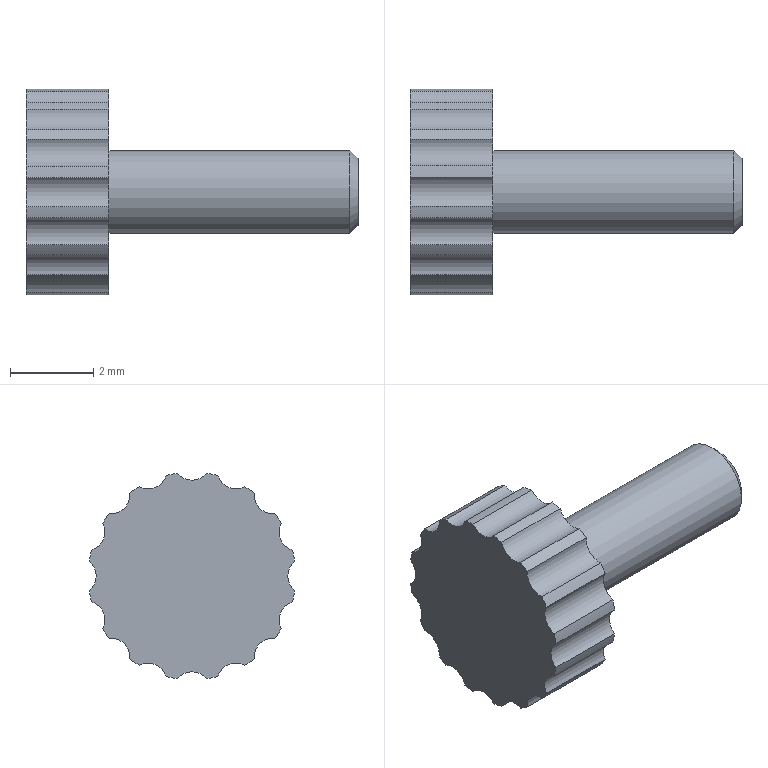Component | NX | 07 | 1 solid | 37 faces | volume 55 mm3 | cylinder 33 | plane 3 | cone 1 | commonest cylinder face diameters 5 x16 0.9 x16 2 x1